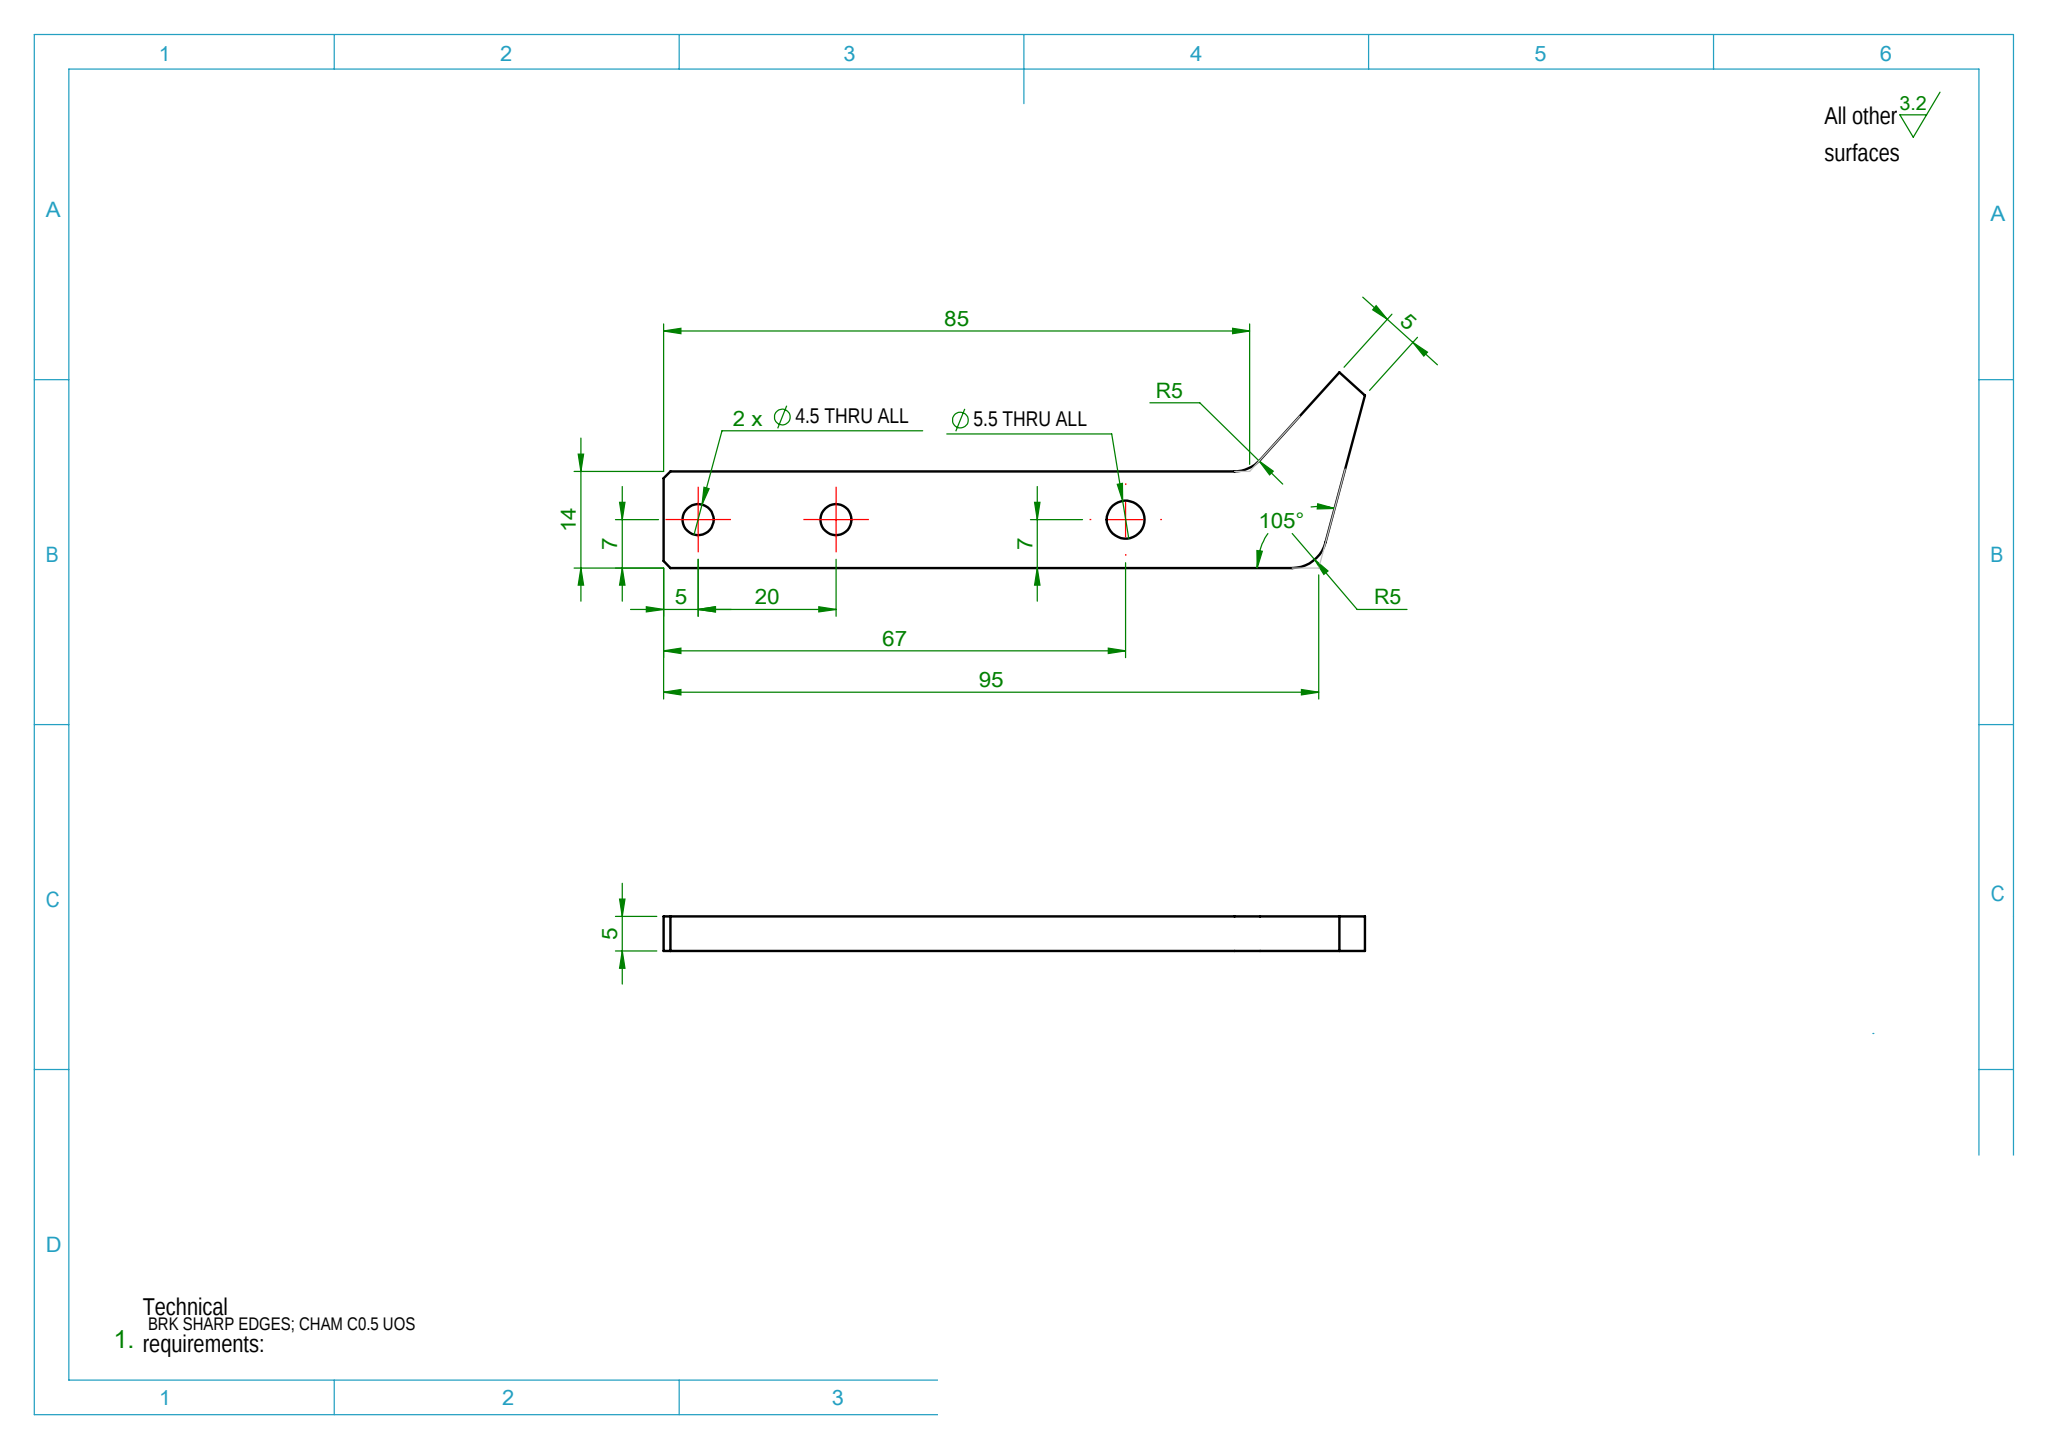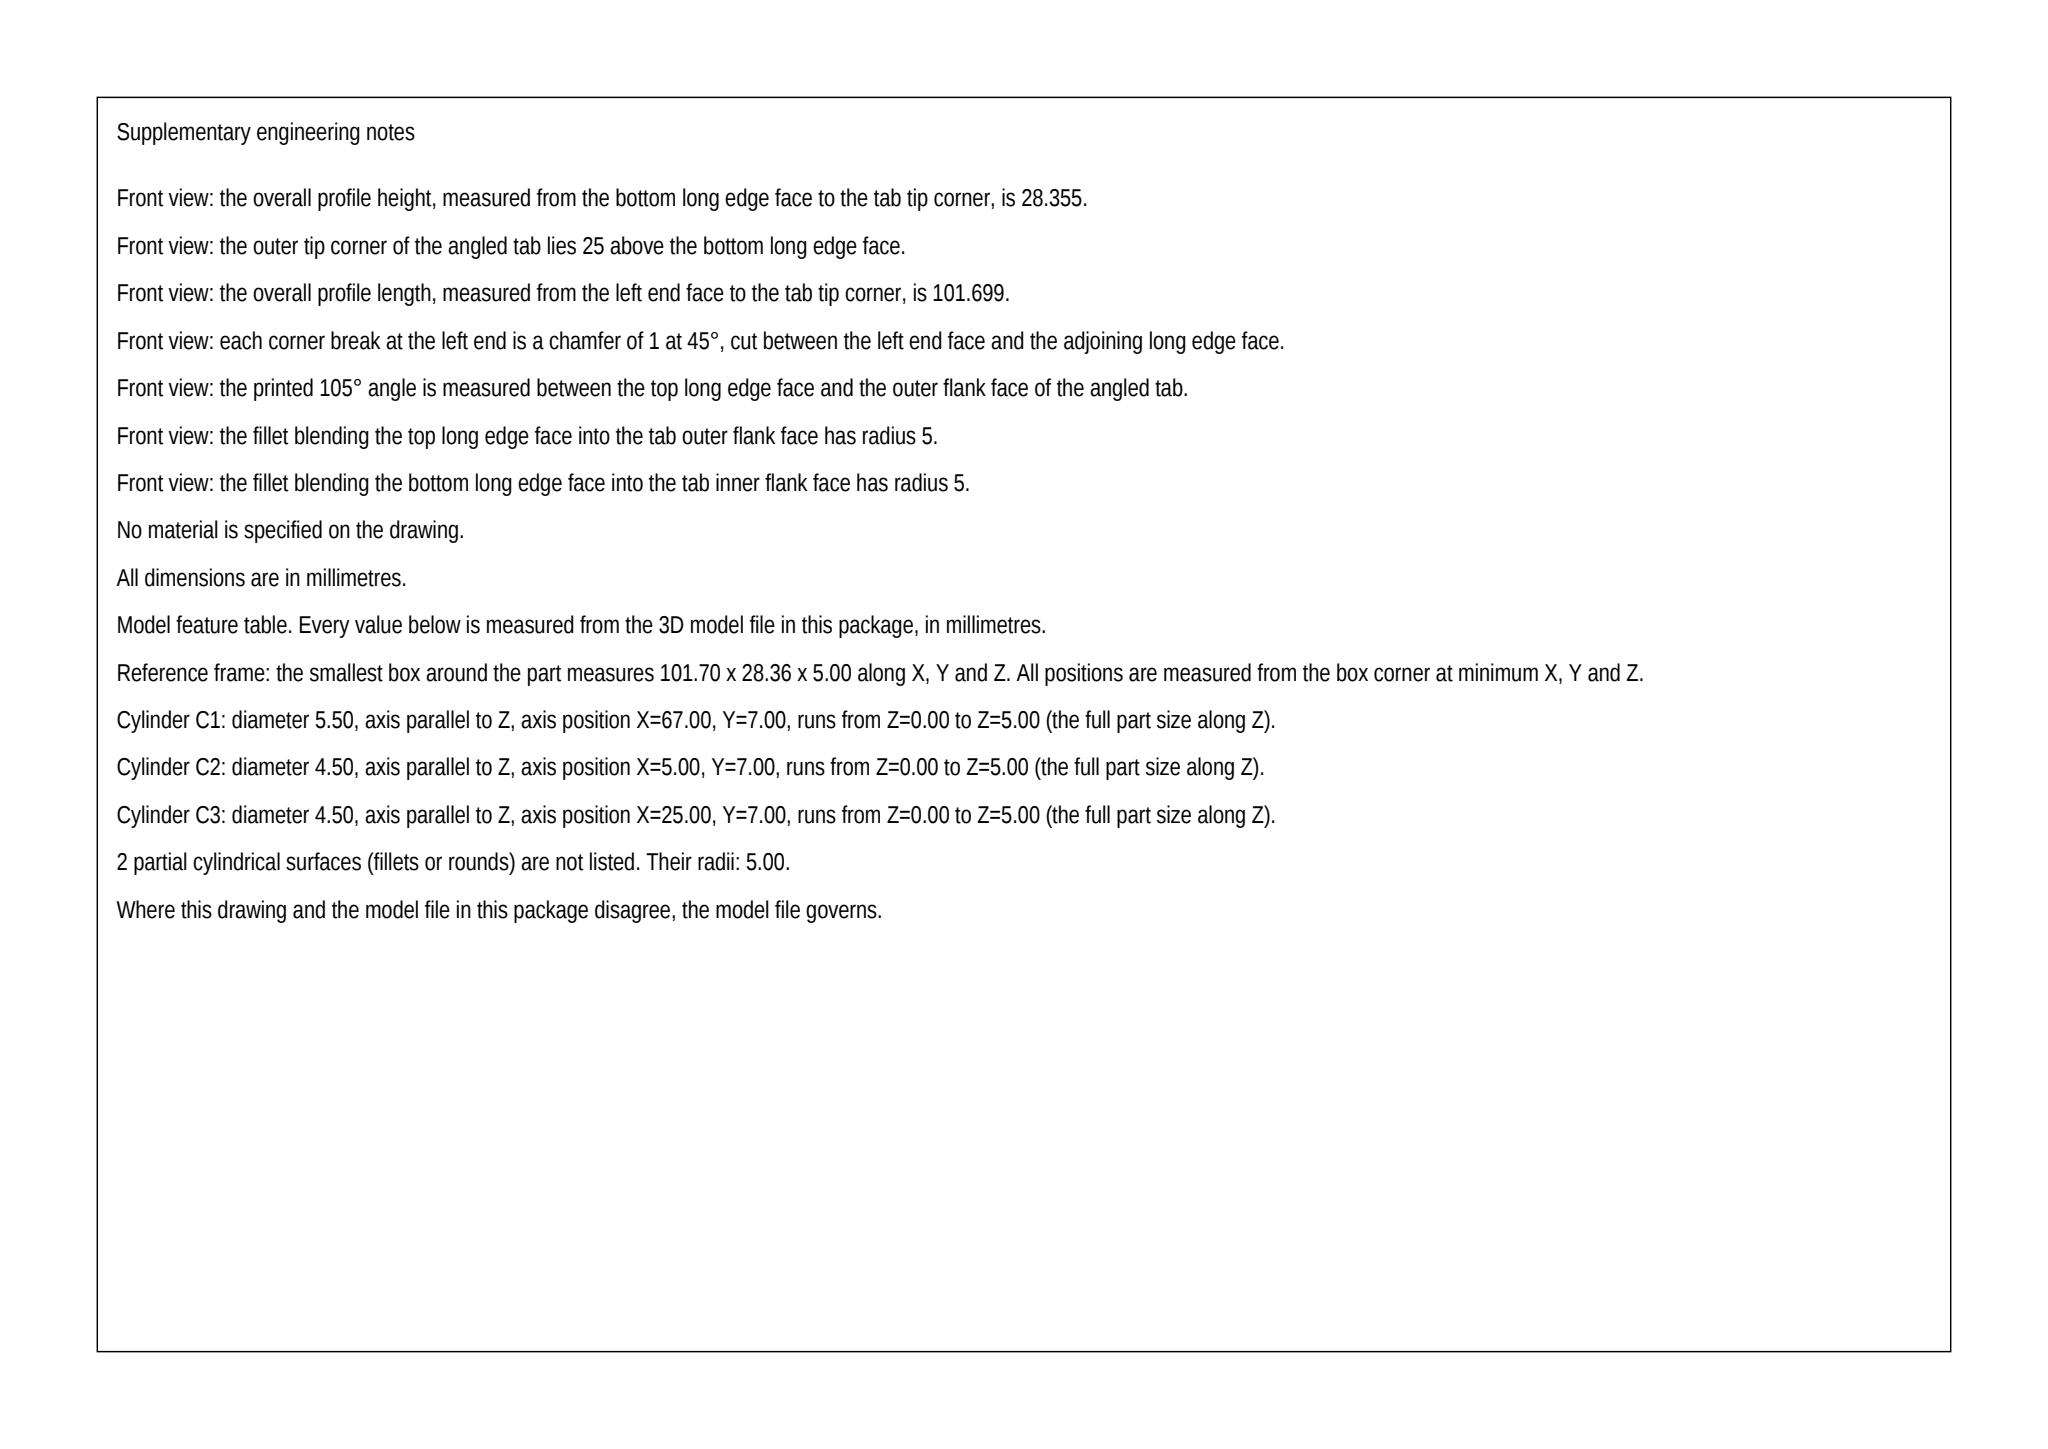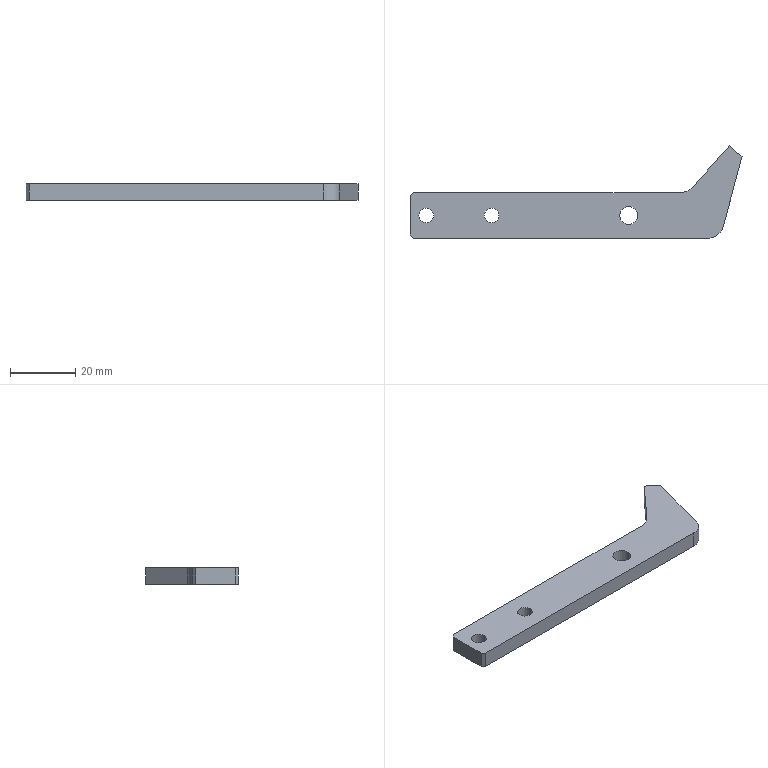Part | SolidWorks | mm | 1 solid | 18 faces | box 101.7 x 28.36 x 5 mm | volume 7108 mm3 | plane 10 | cylinder 8 | commonest cylinder face diameters 4.5 x4 5.5 x2 10 x2
Drawing notes:
OVERALL HT 28.355 FROM BTM EDGE TO TAIL ARM TIP | from the solid: bbox_xyz Y extent = 28.355, plate btm face = plane y=0
OVERALL LG 101.699 FROM LH END FACE | from the solid: bbox_xyz X extent = 101.699, LH end = plane x=0
STEP:
#1=CARTESIAN_POINT('',(69.75,7.,0.));
#2=VERTEX_POINT('',#1);
#3=CARTESIAN_POINT('',(64.25,7.,0.));
#4=VERTEX_POINT('',#3);
#5=CARTESIAN_POINT('',(67.,7.,0.));
#6=DIRECTION('',(0.,0.,-1.));
#7=DIRECTION('',(-1.,0.,0.));
#8=AXIS2_PLACEMENT_3D('',#5,#6,#7);
#9=CIRCLE('',#8,2.75);
#10=EDGE_CURVE('',#2,#4,#9,.T.);
#11=ORIENTED_EDGE('',*,*,#10,.F.);
#12=CARTESIAN_POINT('',(69.75,7.,-5.));
#13=VERTEX_POINT('',#12);
#14=CARTESIAN_POINT('',(69.75,7.,-5.));
#15=DIRECTION('',(0.,0.,-1.));
#16=VECTOR('',#15,1000.);
#17=LINE('',#14,#16);
#18=EDGE_CURVE('',#2,#13,#17,.T.);
#19=ORIENTED_EDGE('',*,*,#18,.T.);
#20=CARTESIAN_POINT('',(64.25,7.,-5.));
#21=VERTEX_POINT('',#20);
#22=CARTESIAN_POINT('',(67.,7.,-5.));
#23=DIRECTION('',(0.,0.,-1.));
#24=DIRECTION('',(-1.,0.,0.));
#25=AXIS2_PLACEMENT_3D('',#22,#23,#24);
#26=CIRCLE('',#25,2.75);
#27=EDGE_CURVE('',#13,#21,#26,.T.);
#28=ORIENTED_EDGE('',*,*,#27,.T.);
#29=CARTESIAN_POINT('',(64.25,7.,-5.));
#30=DIRECTION('',(0.,0.,-1.));
#31=VECTOR('',#30,1000.);
#32=LINE('',#29,#31);
#33=EDGE_CURVE('',#4,#21,#32,.T.);
#34=ORIENTED_EDGE('',*,*,#33,.F.);
#35=EDGE_LOOP('',(#11,#19,#28,#34));
#36=FACE_OUTER_BOUND('',#35,.T.);
#37=CARTESIAN_POINT('',(67.,7.,-5.));
#38=DIRECTION('',(0.,0.,-1.));
#39=DIRECTION('',(-1.,0.,0.));
#40=AXIS2_PLACEMENT_3D('',#37,#38,#39);
#41=CYLINDRICAL_SURFACE('',#40,2.75);
#42=ADVANCED_FACE('',(#36),#41,.F.);
#43=CARTESIAN_POINT('',(2.75,7.,-5.));
#44=VERTEX_POINT('',#43);
#45=CARTESIAN_POINT('',(7.25,7.,-5.));
#46=VERTEX_POINT('',#45);
#47=CARTESIAN_POINT('',(5.,7.,-5.));
#48=DIRECTION('',(0.,0.,1.));
#49=DIRECTION('',(1.,0.,0.));
#50=AXIS2_PLACEMENT_3D('',#47,#48,#49);
#51=CIRCLE('',#50,2.25);
#52=EDGE_CURVE('',#44,#46,#51,.T.);
#53=ORIENTED_EDGE('',*,*,#52,.F.);
#54=CARTESIAN_POINT('',(2.75,7.,-0.));
#55=VERTEX_POINT('',#54);
#56=CARTESIAN_POINT('',(2.75,7.,0.));
#57=DIRECTION('',(0.,0.,1.));
#58=VECTOR('',#57,1000.);
#59=LINE('',#56,#58);
#60=EDGE_CURVE('',#44,#55,#59,.T.);
#61=ORIENTED_EDGE('',*,*,#60,.T.);
#62=CARTESIAN_POINT('',(7.25,7.,-0.));
#63=VERTEX_POINT('',#62);
#64=CARTESIAN_POINT('',(5.,7.,-0.));
#65=DIRECTION('',(0.,0.,1.));
#66=DIRECTION('',(1.,0.,0.));
#67=AXIS2_PLACEMENT_3D('',#64,#65,#66);
#68=CIRCLE('',#67,2.25);
#69=EDGE_CURVE('',#55,#63,#68,.T.);
#70=ORIENTED_EDGE('',*,*,#69,.T.);
#71=CARTESIAN_POINT('',(7.25,7.,0.));
#72=DIRECTION('',(0.,0.,1.));
#73=VECTOR('',#72,1000.);
#74=LINE('',#71,#73);
#75=EDGE_CURVE('',#46,#63,#74,.T.);
#76=ORIENTED_EDGE('',*,*,#75,.F.);
#77=EDGE_LOOP('',(#53,#61,#70,#76));
#78=FACE_OUTER_BOUND('',#77,.T.);
#79=CARTESIAN_POINT('',(5.,7.,0.));
#80=DIRECTION('',(0.,0.,1.));
#81=DIRECTION('',(1.,0.,0.));
#82=AXIS2_PLACEMENT_3D('',#79,#80,#81);
#83=CYLINDRICAL_SURFACE('',#82,2.25);
#84=ADVANCED_FACE('',(#78),#83,.F.);
#85=CARTESIAN_POINT('',(22.75,7.,-5.));
#86=VERTEX_POINT('',#85);
#87=CARTESIAN_POINT('',(27.25,7.,-5.));
#88=VERTEX_POINT('',#87);
#89=CARTESIAN_POINT('',(25.,7.,-5.));
#90=DIRECTION('',(0.,0.,1.));
#91=DIRECTION('',(1.,0.,0.));
#92=AXIS2_PLACEMENT_3D('',#89,#90,#91);
#93=CIRCLE('',#92,2.25);
#94=EDGE_CURVE('',#86,#88,#93,.T.);
#95=ORIENTED_EDGE('',*,*,#94,.F.);
#96=CARTESIAN_POINT('',(22.75,7.,-0.));
#97=VERTEX_POINT('',#96);
#98=CARTESIAN_POINT('',(22.75,7.,0.));
#99=DIRECTION('',(0.,0.,1.));
#100=VECTOR('',#99,1000.);
#101=LINE('',#98,#100);
#102=EDGE_CURVE('',#86,#97,#101,.T.);
#103=ORIENTED_EDGE('',*,*,#102,.T.);
#104=CARTESIAN_POINT('',(27.25,7.,-0.));
#105=VERTEX_POINT('',#104);
#106=CARTESIAN_POINT('',(25.,7.,-0.));
#107=DIRECTION('',(0.,0.,1.));
#108=DIRECTION('',(1.,0.,0.));
#109=AXIS2_PLACEMENT_3D('',#106,#107,#108);
#110=CIRCLE('',#109,2.25);
#111=EDGE_CURVE('',#97,#105,#110,.T.);
#112=ORIENTED_EDGE('',*,*,#111,.T.);
#113=CARTESIAN_POINT('',(27.25,7.,0.));
#114=DIRECTION('',(0.,0.,1.));
#115=VECTOR('',#114,1000.);
#116=LINE('',#113,#115);
#117=EDGE_CURVE('',#88,#105,#116,.T.);
#118=ORIENTED_EDGE('',*,*,#117,.F.);
#119=EDGE_LOOP('',(#95,#103,#112,#118));
#120=FACE_OUTER_BOUND('',#119,.T.);
#121=CARTESIAN_POINT('',(25.,7.,0.));
#122=DIRECTION('',(0.,0.,1.));
#123=DIRECTION('',(1.,0.,0.));
#124=AXIS2_PLACEMENT_3D('',#121,#122,#123);
#125=CYLINDRICAL_SURFACE('',#124,2.25);
#126=ADVANCED_FACE('',(#120),#125,.F.);
#127=CARTESIAN_POINT('',(0.,13.,0.));
#128=VERTEX_POINT('',#127);
#129=CARTESIAN_POINT('',(0.,1.,0.));
#130=VERTEX_POINT('',#129);
#131=CARTESIAN_POINT('',(0.,14.,0.));
#132=DIRECTION('',(0.,-1.,0.));
#133=VECTOR('',#132,1000.);
#134=LINE('',#131,#133);
#135=EDGE_CURVE('',#128,#130,#134,.T.);
#136=ORIENTED_EDGE('',*,*,#135,.F.);
#137=CARTESIAN_POINT('',(0.,13.,-5.));
#138=VERTEX_POINT('',#137);
#139=CARTESIAN_POINT('',(0.,13.,-5.));
#140=DIRECTION('',(0.,0.,-1.));
#141=VECTOR('',#140,1000.);
#142=LINE('',#139,#141);
#143=EDGE_CURVE('',#128,#138,#142,.T.);
#144=ORIENTED_EDGE('',*,*,#143,.T.);
#145=CARTESIAN_POINT('',(0.,1.,-5.));
#146=VERTEX_POINT('',#145);
#147=CARTESIAN_POINT('',(0.,14.,-5.));
#148=DIRECTION('',(0.,-1.,0.));
#149=VECTOR('',#148,1000.);
#150=LINE('',#147,#149);
#151=EDGE_CURVE('',#138,#146,#150,.T.);
#152=ORIENTED_EDGE('',*,*,#151,.T.);
#153=CARTESIAN_POINT('',(0.,1.,-5.));
#154=DIRECTION('',(0.,0.,1.));
#155=VECTOR('',#154,1000.);
#156=LINE('',#153,#155);
#157=EDGE_CURVE('',#146,#130,#156,.T.);
#158=ORIENTED_EDGE('',*,*,#157,.T.);
#159=EDGE_LOOP('',(#136,#144,#152,#158));
#160=FACE_OUTER_BOUND('',#159,.T.);
#161=CARTESIAN_POINT('',(0.,14.,-5.));
#162=DIRECTION('',(-1.,0.,0.));
#163=DIRECTION('',(0.,0.,1.));
#164=AXIS2_PLACEMENT_3D('',#161,#162,#163);
#165=PLANE('',#164);
#166=ADVANCED_FACE('',(#160),#165,.T.);
#167=CARTESIAN_POINT('',(82.781,14.,0.));
#168=VERTEX_POINT('',#167);
#169=CARTESIAN_POINT('',(1.,14.,0.));
#170=VERTEX_POINT('',#169);
#171=CARTESIAN_POINT('',(0.,14.,0.));
#172=DIRECTION('',(-1.,0.,0.));
#173=VECTOR('',#172,1000.);
#174=LINE('',#171,#173);
#175=EDGE_CURVE('',#168,#170,#174,.T.);
#176=ORIENTED_EDGE('',*,*,#175,.F.);
#177=CARTESIAN_POINT('',(82.781,14.,-5.));
#178=VERTEX_POINT('',#177);
#179=CARTESIAN_POINT('',(82.781,14.,-5.));
#180=DIRECTION('',(0.,0.,-1.));
#181=VECTOR('',#180,1000.);
#182=LINE('',#179,#181);
#183=EDGE_CURVE('',#168,#178,#182,.T.);
#184=ORIENTED_EDGE('',*,*,#183,.T.);
#185=CARTESIAN_POINT('',(1.,14.,-5.));
#186=VERTEX_POINT('',#185);
#187=CARTESIAN_POINT('',(0.,14.,-5.));
#188=DIRECTION('',(-1.,0.,0.));
#189=VECTOR('',#188,1000.);
#190=LINE('',#187,#189);
#191=EDGE_CURVE('',#178,#186,#190,.T.);
#192=ORIENTED_EDGE('',*,*,#191,.T.);
#193=CARTESIAN_POINT('',(1.,14.,-5.));
#194=DIRECTION('',(0.,0.,1.));
#195=VECTOR('',#194,1000.);
#196=LINE('',#193,#195);
#197=EDGE_CURVE('',#186,#170,#196,.T.);
#198=ORIENTED_EDGE('',*,*,#197,.T.);
#199=EDGE_LOOP('',(#176,#184,#192,#198));
#200=FACE_OUTER_BOUND('',#199,.T.);
#201=CARTESIAN_POINT('',(0.,14.,-5.));
#202=DIRECTION('',(0.,1.,0.));
#203=DIRECTION('',(0.,0.,1.));
#204=AXIS2_PLACEMENT_3D('',#201,#202,#203);
#205=PLANE('',#204);
#206=ADVANCED_FACE('',(#200),#205,.T.);
#207=CARTESIAN_POINT('',(97.992,28.355,-5.));
#208=VERTEX_POINT('',#207);
#209=CARTESIAN_POINT('',(86.489,15.645,-5.));
#210=VERTEX_POINT('',#209);
#211=CARTESIAN_POINT('',(97.992,28.355,-5.));
#212=DIRECTION('',(-0.671,-0.7414,0.));
#213=VECTOR('',#212,1000.);
#214=LINE('',#211,#213);
#215=EDGE_CURVE('',#208,#210,#214,.T.);
#216=ORIENTED_EDGE('',*,*,#215,.T.);
#217=CARTESIAN_POINT('',(86.489,15.645,0.));
#218=VERTEX_POINT('',#217);
#219=CARTESIAN_POINT('',(86.489,15.645,0.));
#220=DIRECTION('',(0.,0.,1.));
#221=VECTOR('',#220,1000.);
#222=LINE('',#219,#221);
#223=EDGE_CURVE('',#210,#218,#222,.T.);
#224=ORIENTED_EDGE('',*,*,#223,.T.);
#225=CARTESIAN_POINT('',(97.992,28.355,0.));
#226=VERTEX_POINT('',#225);
#227=CARTESIAN_POINT('',(97.992,28.355,0.));
#228=DIRECTION('',(-0.671,-0.7414,0.));
#229=VECTOR('',#228,1000.);
#230=LINE('',#227,#229);
#231=EDGE_CURVE('',#226,#218,#230,.T.);
#232=ORIENTED_EDGE('',*,*,#231,.F.);
#233=CARTESIAN_POINT('',(97.992,28.355,-5.));
#234=DIRECTION('',(0.,0.,1.));
#235=VECTOR('',#234,1000.);
#236=LINE('',#233,#235);
#237=EDGE_CURVE('',#208,#226,#236,.T.);
#238=ORIENTED_EDGE('',*,*,#237,.F.);
#239=EDGE_LOOP('',(#216,#224,#232,#238));
#240=FACE_OUTER_BOUND('',#239,.T.);
#241=CARTESIAN_POINT('',(97.992,28.355,-5.));
#242=DIRECTION('',(-0.7414,0.671,0.));
#243=DIRECTION('',(-0.671,-0.7414,0.));
#244=AXIS2_PLACEMENT_3D('',#241,#242,#243);
#245=PLANE('',#244);
#246=ADVANCED_FACE('',(#240),#245,.T.);
#247=CARTESIAN_POINT('',(101.699,25.,0.));
#248=VERTEX_POINT('',#247);
#249=CARTESIAN_POINT('',(97.992,28.355,0.));
#250=DIRECTION('',(-0.7414,0.671,0.));
#251=VECTOR('',#250,1000.);
#252=LINE('',#249,#251);
#253=EDGE_CURVE('',#248,#226,#252,.T.);
#254=ORIENTED_EDGE('',*,*,#253,.F.);
#255=CARTESIAN_POINT('',(101.699,25.,-5.));
#256=VERTEX_POINT('',#255);
#257=CARTESIAN_POINT('',(101.699,25.,-5.));
#258=DIRECTION('',(0.,0.,1.));
#259=VECTOR('',#258,1000.);
#260=LINE('',#257,#259);
#261=EDGE_CURVE('',#256,#248,#260,.T.);
#262=ORIENTED_EDGE('',*,*,#261,.F.);
#263=CARTESIAN_POINT('',(97.992,28.355,-5.));
#264=DIRECTION('',(-0.7414,0.671,0.));
#265=VECTOR('',#264,1000.);
#266=LINE('',#263,#265);
#267=EDGE_CURVE('',#256,#208,#266,.T.);
#268=ORIENTED_EDGE('',*,*,#267,.T.);
#269=ORIENTED_EDGE('',*,*,#237,.T.);
#270=EDGE_LOOP('',(#254,#262,#268,#269));
#271=FACE_OUTER_BOUND('',#270,.T.);
#272=CARTESIAN_POINT('',(97.992,28.355,-5.));
#273=DIRECTION('',(0.671,0.7414,0.));
#274=DIRECTION('',(-0.7414,0.671,0.));
#275=AXIS2_PLACEMENT_3D('',#272,#273,#274);
#276=PLANE('',#275);
#277=ADVANCED_FACE('',(#271),#276,.T.);
#278=CARTESIAN_POINT('',(95.993,3.706,0.));
#279=VERTEX_POINT('',#278);
#280=CARTESIAN_POINT('',(95.,0.,0.));
#281=DIRECTION('',(0.2588,0.9659,0.));
#282=VECTOR('',#281,1000.);
#283=LINE('',#280,#282);
#284=EDGE_CURVE('',#279,#248,#283,.T.);
#285=ORIENTED_EDGE('',*,*,#284,.F.);
#286=CARTESIAN_POINT('',(95.993,3.706,-5.));
#287=VERTEX_POINT('',#286);
#288=CARTESIAN_POINT('',(95.993,3.706,-5.));
#289=DIRECTION('',(0.,0.,-1.));
#290=VECTOR('',#289,1000.);
#291=LINE('',#288,#290);
#292=EDGE_CURVE('',#279,#287,#291,.T.);
#293=ORIENTED_EDGE('',*,*,#292,.T.);
#294=CARTESIAN_POINT('',(95.,0.,-5.));
#295=DIRECTION('',(0.2588,0.9659,0.));
#296=VECTOR('',#295,1000.);
#297=LINE('',#294,#296);
#298=EDGE_CURVE('',#287,#256,#297,.T.);
#299=ORIENTED_EDGE('',*,*,#298,.T.);
#300=ORIENTED_EDGE('',*,*,#261,.T.);
#301=EDGE_LOOP('',(#285,#293,#299,#300));
#302=FACE_OUTER_BOUND('',#301,.T.);
#303=CARTESIAN_POINT('',(95.,0.,-5.));
#304=DIRECTION('',(0.9659,-0.2588,0.));
#305=DIRECTION('',(0.2588,0.9659,0.));
#306=AXIS2_PLACEMENT_3D('',#303,#304,#305);
#307=PLANE('',#306);
#308=ADVANCED_FACE('',(#302),#307,.T.);
#309=CARTESIAN_POINT('',(1.,0.,-5.));
#310=VERTEX_POINT('',#309);
#311=CARTESIAN_POINT('',(91.163,0.,-5.));
#312=VERTEX_POINT('',#311);
#313=CARTESIAN_POINT('',(0.,0.,-5.));
#314=DIRECTION('',(1.,0.,0.));
#315=VECTOR('',#314,1000.);
#316=LINE('',#313,#315);
#317=EDGE_CURVE('',#310,#312,#316,.T.);
#318=ORIENTED_EDGE('',*,*,#317,.T.);
#319=CARTESIAN_POINT('',(91.163,0.,0.));
#320=VERTEX_POINT('',#319);
#321=CARTESIAN_POINT('',(91.163,0.,-5.));
#322=DIRECTION('',(0.,0.,1.));
#323=VECTOR('',#322,1000.);
#324=LINE('',#321,#323);
#325=EDGE_CURVE('',#312,#320,#324,.T.);
#326=ORIENTED_EDGE('',*,*,#325,.T.);
#327=CARTESIAN_POINT('',(1.,0.,0.));
#328=VERTEX_POINT('',#327);
#329=CARTESIAN_POINT('',(0.,0.,0.));
#330=DIRECTION('',(1.,0.,0.));
#331=VECTOR('',#330,1000.);
#332=LINE('',#329,#331);
#333=EDGE_CURVE('',#328,#320,#332,.T.);
#334=ORIENTED_EDGE('',*,*,#333,.F.);
#335=CARTESIAN_POINT('',(1.,0.,-5.));
#336=DIRECTION('',(0.,0.,-1.));
#337=VECTOR('',#336,1000.);
#338=LINE('',#335,#337);
#339=EDGE_CURVE('',#328,#310,#338,.T.);
#340=ORIENTED_EDGE('',*,*,#339,.T.);
#341=EDGE_LOOP('',(#318,#326,#334,#340));
#342=FACE_OUTER_BOUND('',#341,.T.);
#343=CARTESIAN_POINT('',(0.,0.,-5.));
#344=DIRECTION('',(0.,-1.,0.));
#345=DIRECTION('',(0.,0.,-1.));
#346=AXIS2_PLACEMENT_3D('',#343,#344,#345);
#347=PLANE('',#346);
#348=ADVANCED_FACE('',(#342),#347,.T.);
#349=CARTESIAN_POINT('',(67.,7.,-5.));
#350=DIRECTION('',(0.,0.,-1.));
#351=DIRECTION('',(-1.,0.,0.));
#352=AXIS2_PLACEMENT_3D('',#349,#350,#351);
#353=CIRCLE('',#352,2.75);
#354=EDGE_CURVE('',#21,#13,#353,.T.);
#355=ORIENTED_EDGE('',*,*,#354,.F.);
#356=ORIENTED_EDGE('',*,*,#27,.F.);
#357=EDGE_LOOP('',(#355,#356));
#358=FACE_BOUND('',#357,.T.);
#359=CARTESIAN_POINT('',(5.,7.,-5.));
#360=DIRECTION('',(0.,0.,1.));
#361=DIRECTION('',(1.,0.,0.));
#362=AXIS2_PLACEMENT_3D('',#359,#360,#361);
#363=CIRCLE('',#362,2.25);
#364=EDGE_CURVE('',#46,#44,#363,.T.);
#365=ORIENTED_EDGE('',*,*,#364,.T.);
#366=ORIENTED_EDGE('',*,*,#52,.T.);
#367=EDGE_LOOP('',(#365,#366));
#368=FACE_BOUND('',#367,.T.);
#369=CARTESIAN_POINT('',(25.,7.,-5.));
#370=DIRECTION('',(0.,0.,1.));
#371=DIRECTION('',(1.,0.,0.));
#372=AXIS2_PLACEMENT_3D('',#369,#370,#371);
#373=CIRCLE('',#372,2.25);
#374=EDGE_CURVE('',#88,#86,#373,.T.);
#375=ORIENTED_EDGE('',*,*,#374,.T.);
#376=ORIENTED_EDGE('',*,*,#94,.T.);
#377=EDGE_LOOP('',(#375,#376));
#378=FACE_BOUND('',#377,.T.);
#379=ORIENTED_EDGE('',*,*,#298,.F.);
#380=CARTESIAN_POINT('',(91.163,5.,-5.));
#381=DIRECTION('',(0.,0.,-1.));
#382=DIRECTION('',(1.,0.,0.));
#383=AXIS2_PLACEMENT_3D('',#380,#381,#382);
#384=CIRCLE('',#383,5.);
#385=EDGE_CURVE('',#287,#312,#384,.T.);
#386=ORIENTED_EDGE('',*,*,#385,.T.);
#387=ORIENTED_EDGE('',*,*,#317,.F.);
#388=CARTESIAN_POINT('',(0.,1.,-5.));
#389=DIRECTION('',(-0.7071,0.7071,0.));
#390=VECTOR('',#389,1000.);
#391=LINE('',#388,#390);
#392=EDGE_CURVE('',#310,#146,#391,.T.);
#393=ORIENTED_EDGE('',*,*,#392,.T.);
#394=ORIENTED_EDGE('',*,*,#151,.F.);
#395=CARTESIAN_POINT('',(1.,14.,-5.));
#396=DIRECTION('',(0.7071,0.7071,0.));
#397=VECTOR('',#396,1000.);
#398=LINE('',#395,#397);
#399=EDGE_CURVE('',#138,#186,#398,.T.);
#400=ORIENTED_EDGE('',*,*,#399,.T.);
#401=ORIENTED_EDGE('',*,*,#191,.F.);
#402=CARTESIAN_POINT('',(82.781,19.,-5.));
#403=DIRECTION('',(0.,0.,1.));
#404=DIRECTION('',(1.,0.,0.));
#405=AXIS2_PLACEMENT_3D('',#402,#403,#404);
#406=CIRCLE('',#405,5.);
#407=EDGE_CURVE('',#178,#210,#406,.T.);
#408=ORIENTED_EDGE('',*,*,#407,.T.);
#409=ORIENTED_EDGE('',*,*,#215,.F.);
#410=ORIENTED_EDGE('',*,*,#267,.F.);
#411=EDGE_LOOP('',(#379,#386,#387,#393,#394,#400,#401,#408,#409,#410));
#412=FACE_OUTER_BOUND('',#411,.T.);
#413=CARTESIAN_POINT('',(0.,0.,-5.));
#414=DIRECTION('',(0.,0.,1.));
#415=DIRECTION('',(1.,0.,0.));
#416=AXIS2_PLACEMENT_3D('',#413,#414,#415);
#417=PLANE('',#416);
#418=ADVANCED_FACE('',(#358,#368,#378,#412),#417,.F.);
#419=CARTESIAN_POINT('',(67.,7.,0.));
#420=DIRECTION('',(0.,0.,-1.));
#421=DIRECTION('',(-1.,0.,0.));
#422=AXIS2_PLACEMENT_3D('',#419,#420,#421);
#423=CIRCLE('',#422,2.75);
#424=EDGE_CURVE('',#4,#2,#423,.T.);
#425=ORIENTED_EDGE('',*,*,#424,.T.);
#426=ORIENTED_EDGE('',*,*,#10,.T.);
#427=EDGE_LOOP('',(#425,#426));
#428=FACE_BOUND('',#427,.T.);
#429=CARTESIAN_POINT('',(5.,7.,-0.));
#430=DIRECTION('',(0.,0.,1.));
#431=DIRECTION('',(1.,0.,0.));
#432=AXIS2_PLACEMENT_3D('',#429,#430,#431);
#433=CIRCLE('',#432,2.25);
#434=EDGE_CURVE('',#63,#55,#433,.T.);
#435=ORIENTED_EDGE('',*,*,#434,.F.);
#436=ORIENTED_EDGE('',*,*,#69,.F.);
#437=EDGE_LOOP('',(#435,#436));
#438=FACE_BOUND('',#437,.T.);
#439=CARTESIAN_POINT('',(25.,7.,-0.));
#440=DIRECTION('',(0.,0.,1.));
#441=DIRECTION('',(1.,0.,0.));
#442=AXIS2_PLACEMENT_3D('',#439,#440,#441);
#443=CIRCLE('',#442,2.25);
#444=EDGE_CURVE('',#105,#97,#443,.T.);
#445=ORIENTED_EDGE('',*,*,#444,.F.);
#446=ORIENTED_EDGE('',*,*,#111,.F.);
#447=EDGE_LOOP('',(#445,#446));
#448=FACE_BOUND('',#447,.T.);
#449=ORIENTED_EDGE('',*,*,#333,.T.);
#450=CARTESIAN_POINT('',(91.163,5.,0.));
#451=DIRECTION('',(0.,0.,1.));
#452=DIRECTION('',(1.,0.,0.));
#453=AXIS2_PLACEMENT_3D('',#450,#451,#452);
#454=CIRCLE('',#453,5.);
#455=EDGE_CURVE('',#320,#279,#454,.T.);
#456=ORIENTED_EDGE('',*,*,#455,.T.);
#457=ORIENTED_EDGE('',*,*,#284,.T.);
#458=ORIENTED_EDGE('',*,*,#253,.T.);
#459=ORIENTED_EDGE('',*,*,#231,.T.);
#460=CARTESIAN_POINT('',(82.781,19.,0.));
#461=DIRECTION('',(0.,0.,-1.));
#462=DIRECTION('',(1.,-0.,0.));
#463=AXIS2_PLACEMENT_3D('',#460,#461,#462);
#464=CIRCLE('',#463,5.);
#465=EDGE_CURVE('',#218,#168,#464,.T.);
#466=ORIENTED_EDGE('',*,*,#465,.T.);
#467=ORIENTED_EDGE('',*,*,#175,.T.);
#468=CARTESIAN_POINT('',(-6.5,6.5,0.));
#469=DIRECTION('',(-0.7071,-0.7071,0.));
#470=VECTOR('',#469,1000.);
#471=LINE('',#468,#470);
#472=EDGE_CURVE('',#170,#128,#471,.T.);
#473=ORIENTED_EDGE('',*,*,#472,.T.);
#474=ORIENTED_EDGE('',*,*,#135,.T.);
#475=CARTESIAN_POINT('',(0.5,0.5,0.));
#476=DIRECTION('',(0.7071,-0.7071,0.));
#477=VECTOR('',#476,1000.);
#478=LINE('',#475,#477);
#479=EDGE_CURVE('',#130,#328,#478,.T.);
#480=ORIENTED_EDGE('',*,*,#479,.T.);
#481=EDGE_LOOP('',(#449,#456,#457,#458,#459,#466,#467,#473,#474,#480));
#482=FACE_OUTER_BOUND('',#481,.T.);
#483=CARTESIAN_POINT('',(0.,0.,0.));
#484=DIRECTION('',(0.,0.,1.));
#485=DIRECTION('',(1.,0.,0.));
#486=AXIS2_PLACEMENT_3D('',#483,#484,#485);
#487=PLANE('',#486);
#488=ADVANCED_FACE('',(#428,#438,#448,#482),#487,.T.);
#489=ORIENTED_EDGE('',*,*,#399,.F.);
#490=ORIENTED_EDGE('',*,*,#143,.F.);
#491=ORIENTED_EDGE('',*,*,#472,.F.);
#492=ORIENTED_EDGE('',*,*,#197,.F.);
#493=EDGE_LOOP('',(#489,#490,#491,#492));
#494=FACE_OUTER_BOUND('',#493,.T.);
#495=CARTESIAN_POINT('',(1.,14.,-5.));
#496=DIRECTION('',(0.7071,-0.7071,0.));
#497=DIRECTION('',(0.,0.,1.));
#498=AXIS2_PLACEMENT_3D('',#495,#496,#497);
#499=PLANE('',#498);
#500=ADVANCED_FACE('',(#494),#499,.F.);
#501=ORIENTED_EDGE('',*,*,#392,.F.);
#502=ORIENTED_EDGE('',*,*,#339,.F.);
#503=ORIENTED_EDGE('',*,*,#479,.F.);
#504=ORIENTED_EDGE('',*,*,#157,.F.);
#505=EDGE_LOOP('',(#501,#502,#503,#504));
#506=FACE_OUTER_BOUND('',#505,.T.);
#507=CARTESIAN_POINT('',(0.,1.,-5.));
#508=DIRECTION('',(0.7071,0.7071,0.));
#509=DIRECTION('',(0.,0.,1.));
#510=AXIS2_PLACEMENT_3D('',#507,#508,#509);
#511=PLANE('',#510);
#512=ADVANCED_FACE('',(#506),#511,.F.);
#513=ORIENTED_EDGE('',*,*,#102,.F.);
#514=ORIENTED_EDGE('',*,*,#374,.F.);
#515=ORIENTED_EDGE('',*,*,#117,.T.);
#516=ORIENTED_EDGE('',*,*,#444,.T.);
#517=EDGE_LOOP('',(#513,#514,#515,#516));
#518=FACE_OUTER_BOUND('',#517,.T.);
#519=CARTESIAN_POINT('',(25.,7.,0.));
#520=DIRECTION('',(0.,0.,1.));
#521=DIRECTION('',(1.,0.,0.));
#522=AXIS2_PLACEMENT_3D('',#519,#520,#521);
#523=CYLINDRICAL_SURFACE('',#522,2.25);
#524=ADVANCED_FACE('',(#518),#523,.F.);
#525=ORIENTED_EDGE('',*,*,#60,.F.);
#526=ORIENTED_EDGE('',*,*,#364,.F.);
#527=ORIENTED_EDGE('',*,*,#75,.T.);
#528=ORIENTED_EDGE('',*,*,#434,.T.);
#529=EDGE_LOOP('',(#525,#526,#527,#528));
#530=FACE_OUTER_BOUND('',#529,.T.);
#531=CARTESIAN_POINT('',(5.,7.,0.));
#532=DIRECTION('',(0.,0.,1.));
#533=DIRECTION('',(1.,0.,0.));
#534=AXIS2_PLACEMENT_3D('',#531,#532,#533);
#535=CYLINDRICAL_SURFACE('',#534,2.25);
#536=ADVANCED_FACE('',(#530),#535,.F.);
#537=ORIENTED_EDGE('',*,*,#385,.F.);
#538=ORIENTED_EDGE('',*,*,#292,.F.);
#539=ORIENTED_EDGE('',*,*,#455,.F.);
#540=ORIENTED_EDGE('',*,*,#325,.F.);
#541=EDGE_LOOP('',(#537,#538,#539,#540));
#542=FACE_OUTER_BOUND('',#541,.T.);
#543=CARTESIAN_POINT('',(91.163,5.,-5.));
#544=DIRECTION('',(0.,0.,1.));
#545=DIRECTION('',(1.,0.,0.));
#546=AXIS2_PLACEMENT_3D('',#543,#544,#545);
#547=CYLINDRICAL_SURFACE('',#546,5.);
#548=ADVANCED_FACE('',(#542),#547,.T.);
#549=ORIENTED_EDGE('',*,*,#407,.F.);
#550=ORIENTED_EDGE('',*,*,#183,.F.);
#551=ORIENTED_EDGE('',*,*,#465,.F.);
#552=ORIENTED_EDGE('',*,*,#223,.F.);
#553=EDGE_LOOP('',(#549,#550,#551,#552));
#554=FACE_OUTER_BOUND('',#553,.T.);
#555=CARTESIAN_POINT('',(82.781,19.,-5.));
#556=DIRECTION('',(0.,0.,-1.));
#557=DIRECTION('',(-1.,0.,0.));
#558=AXIS2_PLACEMENT_3D('',#555,#556,#557);
#559=CYLINDRICAL_SURFACE('',#558,5.);
#560=ADVANCED_FACE('',(#554),#559,.F.);
#561=ORIENTED_EDGE('',*,*,#18,.F.);
#562=ORIENTED_EDGE('',*,*,#424,.F.);
#563=ORIENTED_EDGE('',*,*,#33,.T.);
#564=ORIENTED_EDGE('',*,*,#354,.T.);
#565=EDGE_LOOP('',(#561,#562,#563,#564));
#566=FACE_OUTER_BOUND('',#565,.T.);
#567=CARTESIAN_POINT('',(67.,7.,-5.));
#568=DIRECTION('',(0.,0.,-1.));
#569=DIRECTION('',(-1.,0.,0.));
#570=AXIS2_PLACEMENT_3D('',#567,#568,#569);
#571=CYLINDRICAL_SURFACE('',#570,2.75);
#572=ADVANCED_FACE('',(#566),#571,.F.);
#573=CLOSED_SHELL('',(#42,#84,#126,#166,#206,#246,#277,#308,#348,#418,#488,#500,#512,#524,#536,#548,#560,#572));
#574=MANIFOLD_SOLID_BREP('',#573);
#575=CARTESIAN_POINT('',(0.,0.,0.));
#576=DIRECTION('',(0.,0.,1.));
#577=DIRECTION('',(1.,0.,0.));
#578=AXIS2_PLACEMENT_3D('',#575,#576,#577);
#579=(LENGTH_UNIT()NAMED_UNIT(*)SI_UNIT(.MILLI.,.METRE.));
#580=UNCERTAINTY_MEASURE_WITH_UNIT(LENGTH_MEASURE(0.00001),#579,'','');
#581=(NAMED_UNIT(*)PLANE_ANGLE_UNIT()SI_UNIT($,.RADIAN.));
#582=(NAMED_UNIT(*)SI_UNIT($,.STERADIAN.)SOLID_ANGLE_UNIT());
#583=(GEOMETRIC_REPRESENTATION_CONTEXT(3)GLOBAL_UNCERTAINTY_ASSIGNED_CONTEXT((#580))GLOBAL_UNIT_ASSIGNED_CONTEXT((#579,#581,#582))REPRESENTATION_CONTEXT('',''));
#584=ADVANCED_BREP_SHAPE_REPRESENTATION('',(#574,#578),#583);